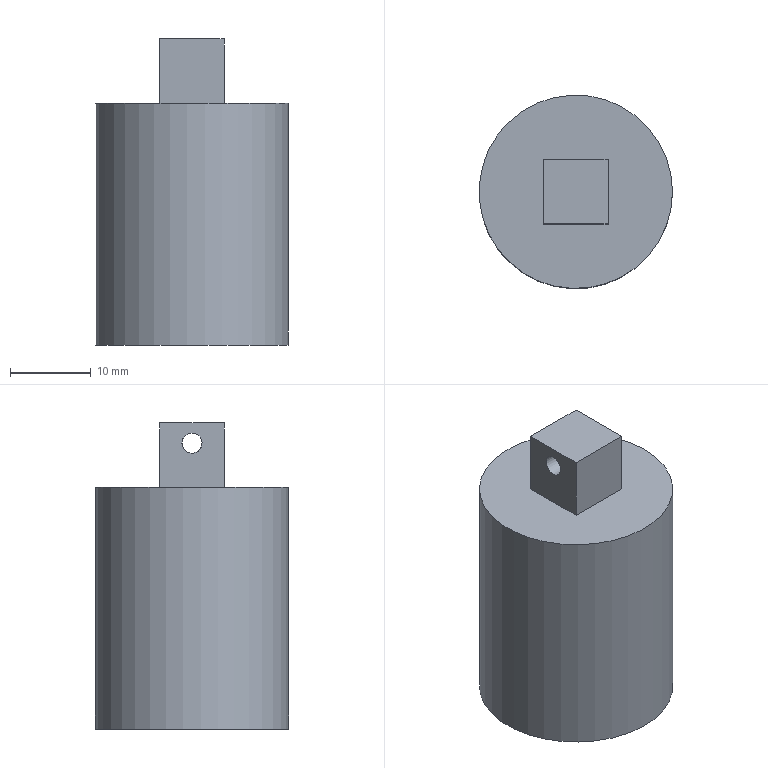Component | NX | ROBOT_ARM_BASE | 1 solid | 9 faces | box 24 x 24 x 38 mm | volume 14044 mm3 | plane 7 | cylinder 2 | commonest cylinder face diameters 24 x1 2.5 x1
STEP:
#1=CARTESIAN_POINT('',(0.,0.,0.));
#2=DIRECTION('',(0.,0.,1.));
#3=DIRECTION('',(1.,0.,0.));
#4=AXIS2_PLACEMENT_3D('',#1,#2,#3);
#5=CARTESIAN_POINT('',(23.471,13.498,36.));
#6=VERTEX_POINT('',#5);
#7=CARTESIAN_POINT('',(11.471,13.498,36.));
#8=DIRECTION('',(0.,0.,-1.));
#9=DIRECTION('',(1.,0.,0.));
#10=AXIS2_PLACEMENT_3D('',#7,#8,#9);
#11=CIRCLE('',#10,12.);
#12=CARTESIAN_POINT('',(11.471,13.498,36.));
#13=DIRECTION('',(0.,0.,-1.));
#14=DIRECTION('',(-1.,0.,0.));
#15=AXIS2_PLACEMENT_3D('',#12,#13,#14);
#16=PLANE('',#15);
#17=CARTESIAN_POINT('',(0.,0.));
#18=DIRECTION('',(-1.,0.));
#19=AXIS2_PLACEMENT_2D('',#17,#18);
#20=CIRCLE('',#19,12.);
#21=(GEOMETRIC_REPRESENTATION_CONTEXT(2)PARAMETRIC_REPRESENTATION_CONTEXT()REPRESENTATION_CONTEXT('',''));
#22=DEFINITIONAL_REPRESENTATION('',(#20),#21);
#23=PCURVE('',#16,#22);
#24=CARTESIAN_POINT('',(11.471,13.498,6.));
#25=DIRECTION('',(0.,0.,1.));
#26=DIRECTION('',(1.,0.,0.));
#27=AXIS2_PLACEMENT_3D('',#24,#25,#26);
#28=CYLINDRICAL_SURFACE('',#27,12.);
#29=CARTESIAN_POINT('',(6.283,30.));
#30=DIRECTION('',(-1.,0.));
#31=VECTOR('',#30,1.);
#32=LINE('',#29,#31);
#33=(GEOMETRIC_REPRESENTATION_CONTEXT(2)PARAMETRIC_REPRESENTATION_CONTEXT()REPRESENTATION_CONTEXT('',''));
#34=DEFINITIONAL_REPRESENTATION('',(#32),#33);
#35=PCURVE('',#28,#34);
#36=SURFACE_CURVE('',#11,(#23,#35),.PCURVE_S1.);
#37=EDGE_CURVE('',#6,#6,#36,.T.);
#38=ORIENTED_EDGE('',*,*,#37,.F.);
#39=EDGE_LOOP('',(#38));
#40=FACE_BOUND('',#39,.T.);
#41=CARTESIAN_POINT('',(7.471,17.498,36.));
#42=VERTEX_POINT('',#41);
#43=CARTESIAN_POINT('',(7.471,9.498,36.));
#44=VERTEX_POINT('',#43);
#45=CARTESIAN_POINT('',(7.471,17.498,36.));
#46=DIRECTION('',(-0.,-1.,0.));
#47=VECTOR('',#46,1.);
#48=LINE('',#45,#47);
#49=CARTESIAN_POINT('',(4.,4.));
#50=DIRECTION('',(0.,-1.));
#51=VECTOR('',#50,1.);
#52=LINE('',#49,#51);
#53=(GEOMETRIC_REPRESENTATION_CONTEXT(2)PARAMETRIC_REPRESENTATION_CONTEXT()REPRESENTATION_CONTEXT('',''));
#54=DEFINITIONAL_REPRESENTATION('',(#52),#53);
#55=PCURVE('',#16,#54);
#56=CARTESIAN_POINT('',(7.471,17.498,44.));
#57=DIRECTION('',(1.,-0.,0.));
#58=DIRECTION('',(0.,1.,0.));
#59=AXIS2_PLACEMENT_3D('',#56,#57,#58);
#60=PLANE('',#59);
#61=CARTESIAN_POINT('',(0.,-8.));
#62=DIRECTION('',(-1.,0.));
#63=VECTOR('',#62,1.);
#64=LINE('',#61,#63);
#65=(GEOMETRIC_REPRESENTATION_CONTEXT(2)PARAMETRIC_REPRESENTATION_CONTEXT()REPRESENTATION_CONTEXT('',''));
#66=DEFINITIONAL_REPRESENTATION('',(#64),#65);
#67=PCURVE('',#60,#66);
#68=SURFACE_CURVE('',#48,(#55,#67),.PCURVE_S1.);
#69=EDGE_CURVE('',#42,#44,#68,.T.);
#70=ORIENTED_EDGE('',*,*,#69,.F.);
#71=CARTESIAN_POINT('',(15.471,17.498,36.));
#72=VERTEX_POINT('',#71);
#73=CARTESIAN_POINT('',(15.471,17.498,36.));
#74=DIRECTION('',(-1.,0.,0.));
#75=VECTOR('',#74,1.);
#76=LINE('',#73,#75);
#77=CARTESIAN_POINT('',(-4.,4.));
#78=DIRECTION('',(1.,0.));
#79=VECTOR('',#78,1.);
#80=LINE('',#77,#79);
#81=(GEOMETRIC_REPRESENTATION_CONTEXT(2)PARAMETRIC_REPRESENTATION_CONTEXT()REPRESENTATION_CONTEXT('',''));
#82=DEFINITIONAL_REPRESENTATION('',(#80),#81);
#83=PCURVE('',#16,#82);
#84=CARTESIAN_POINT('',(15.471,17.498,44.));
#85=DIRECTION('',(-0.,-1.,0.));
#86=DIRECTION('',(1.,-0.,0.));
#87=AXIS2_PLACEMENT_3D('',#84,#85,#86);
#88=PLANE('',#87);
#89=CARTESIAN_POINT('',(0.,-8.));
#90=DIRECTION('',(-1.,0.));
#91=VECTOR('',#90,1.);
#92=LINE('',#89,#91);
#93=(GEOMETRIC_REPRESENTATION_CONTEXT(2)PARAMETRIC_REPRESENTATION_CONTEXT()REPRESENTATION_CONTEXT('',''));
#94=DEFINITIONAL_REPRESENTATION('',(#92),#93);
#95=PCURVE('',#88,#94);
#96=SURFACE_CURVE('',#76,(#83,#95),.PCURVE_S1.);
#97=EDGE_CURVE('',#72,#42,#96,.T.);
#98=ORIENTED_EDGE('',*,*,#97,.F.);
#99=CARTESIAN_POINT('',(15.471,9.498,36.));
#100=VERTEX_POINT('',#99);
#101=CARTESIAN_POINT('',(15.471,9.498,36.));
#102=DIRECTION('',(0.,1.,0.));
#103=VECTOR('',#102,1.);
#104=LINE('',#101,#103);
#105=CARTESIAN_POINT('',(-4.,-4.));
#106=DIRECTION('',(0.,1.));
#107=VECTOR('',#106,1.);
#108=LINE('',#105,#107);
#109=(GEOMETRIC_REPRESENTATION_CONTEXT(2)PARAMETRIC_REPRESENTATION_CONTEXT()REPRESENTATION_CONTEXT('',''));
#110=DEFINITIONAL_REPRESENTATION('',(#108),#109);
#111=PCURVE('',#16,#110);
#112=CARTESIAN_POINT('',(15.471,9.498,44.));
#113=DIRECTION('',(-1.,0.,0.));
#114=DIRECTION('',(0.,0.,1.));
#115=AXIS2_PLACEMENT_3D('',#112,#113,#114);
#116=PLANE('',#115);
#117=CARTESIAN_POINT('',(-8.,0.));
#118=DIRECTION('',(0.,1.));
#119=VECTOR('',#118,1.);
#120=LINE('',#117,#119);
#121=(GEOMETRIC_REPRESENTATION_CONTEXT(2)PARAMETRIC_REPRESENTATION_CONTEXT()REPRESENTATION_CONTEXT('',''));
#122=DEFINITIONAL_REPRESENTATION('',(#120),#121);
#123=PCURVE('',#116,#122);
#124=SURFACE_CURVE('',#104,(#111,#123),.PCURVE_S1.);
#125=EDGE_CURVE('',#100,#72,#124,.T.);
#126=ORIENTED_EDGE('',*,*,#125,.F.);
#127=CARTESIAN_POINT('',(7.471,9.498,36.));
#128=DIRECTION('',(1.,0.,0.));
#129=VECTOR('',#128,1.);
#130=LINE('',#127,#129);
#131=CARTESIAN_POINT('',(4.,-4.));
#132=DIRECTION('',(-1.,0.));
#133=VECTOR('',#132,1.);
#134=LINE('',#131,#133);
#135=(GEOMETRIC_REPRESENTATION_CONTEXT(2)PARAMETRIC_REPRESENTATION_CONTEXT()REPRESENTATION_CONTEXT('',''));
#136=DEFINITIONAL_REPRESENTATION('',(#134),#135);
#137=PCURVE('',#16,#136);
#138=CARTESIAN_POINT('',(7.471,9.498,44.));
#139=DIRECTION('',(0.,1.,0.));
#140=DIRECTION('',(0.,0.,1.));
#141=AXIS2_PLACEMENT_3D('',#138,#139,#140);
#142=PLANE('',#141);
#143=CARTESIAN_POINT('',(-8.,0.));
#144=DIRECTION('',(0.,1.));
#145=VECTOR('',#144,1.);
#146=LINE('',#143,#145);
#147=(GEOMETRIC_REPRESENTATION_CONTEXT(2)PARAMETRIC_REPRESENTATION_CONTEXT()REPRESENTATION_CONTEXT('',''));
#148=DEFINITIONAL_REPRESENTATION('',(#146),#147);
#149=PCURVE('',#142,#148);
#150=SURFACE_CURVE('',#130,(#137,#149),.PCURVE_S1.);
#151=EDGE_CURVE('',#44,#100,#150,.T.);
#152=ORIENTED_EDGE('',*,*,#151,.F.);
#153=EDGE_LOOP('',(#70,#98,#126,#152));
#154=FACE_BOUND('',#153,.T.);
#155=ADVANCED_FACE('',(#40,#154),#16,.F.);
#156=CARTESIAN_POINT('',(23.471,13.498,6.));
#157=VERTEX_POINT('',#156);
#158=CARTESIAN_POINT('',(11.471,13.498,6.));
#159=DIRECTION('',(0.,0.,-1.));
#160=DIRECTION('',(1.,0.,0.));
#161=AXIS2_PLACEMENT_3D('',#158,#159,#160);
#162=CIRCLE('',#161,12.);
#163=CARTESIAN_POINT('',(6.283,0.));
#164=DIRECTION('',(-1.,0.));
#165=VECTOR('',#164,1.);
#166=LINE('',#163,#165);
#167=(GEOMETRIC_REPRESENTATION_CONTEXT(2)PARAMETRIC_REPRESENTATION_CONTEXT()REPRESENTATION_CONTEXT('',''));
#168=DEFINITIONAL_REPRESENTATION('',(#166),#167);
#169=PCURVE('',#28,#168);
#170=CARTESIAN_POINT('',(11.471,13.498,6.));
#171=DIRECTION('',(0.,0.,-1.));
#172=DIRECTION('',(-1.,0.,0.));
#173=AXIS2_PLACEMENT_3D('',#170,#171,#172);
#174=PLANE('',#173);
#175=CARTESIAN_POINT('',(0.,0.));
#176=DIRECTION('',(-1.,0.));
#177=AXIS2_PLACEMENT_2D('',#175,#176);
#178=CIRCLE('',#177,12.);
#179=(GEOMETRIC_REPRESENTATION_CONTEXT(2)PARAMETRIC_REPRESENTATION_CONTEXT()REPRESENTATION_CONTEXT('',''));
#180=DEFINITIONAL_REPRESENTATION('',(#178),#179);
#181=PCURVE('',#174,#180);
#182=SURFACE_CURVE('',#162,(#169,#181),.PCURVE_S1.);
#183=EDGE_CURVE('',#157,#157,#182,.T.);
#184=ORIENTED_EDGE('',*,*,#183,.F.);
#185=CARTESIAN_POINT('',(23.471,13.498,6.));
#186=CARTESIAN_POINT('',(23.471,13.498,36.));
#187=B_SPLINE_CURVE_WITH_KNOTS('',1,(#185,#186),.UNSPECIFIED.,.F.,.F.,(2,2),(0.,30.),.PIECEWISE_BEZIER_KNOTS.);
#188=CARTESIAN_POINT('',(6.283,0.));
#189=DIRECTION('',(0.,1.));
#190=VECTOR('',#189,1.);
#191=LINE('',#188,#190);
#192=(GEOMETRIC_REPRESENTATION_CONTEXT(2)PARAMETRIC_REPRESENTATION_CONTEXT()REPRESENTATION_CONTEXT('',''));
#193=DEFINITIONAL_REPRESENTATION('',(#191),#192);
#194=PCURVE('',#28,#193);
#195=CARTESIAN_POINT('',(0.,0.));
#196=DIRECTION('',(0.,1.));
#197=VECTOR('',#196,1.);
#198=LINE('',#195,#197);
#199=(GEOMETRIC_REPRESENTATION_CONTEXT(2)PARAMETRIC_REPRESENTATION_CONTEXT()REPRESENTATION_CONTEXT('',''));
#200=DEFINITIONAL_REPRESENTATION('',(#198),#199);
#201=PCURVE('',#28,#200);
#202=SEAM_CURVE('',#187,(#194,#201),.PCURVE_S1.);
#203=EDGE_CURVE('',#157,#6,#202,.T.);
#204=ORIENTED_EDGE('',*,*,#203,.T.);
#205=ORIENTED_EDGE('',*,*,#37,.T.);
#206=ORIENTED_EDGE('',*,*,#203,.F.);
#207=EDGE_LOOP('',(#184,#204,#205,#206));
#208=FACE_BOUND('',#207,.T.);
#209=ADVANCED_FACE('',(#208),#28,.T.);
#210=ORIENTED_EDGE('',*,*,#183,.T.);
#211=EDGE_LOOP('',(#210));
#212=FACE_BOUND('',#211,.T.);
#213=ADVANCED_FACE('',(#212),#174,.T.);
#214=CARTESIAN_POINT('',(7.471,14.748,41.5));
#215=VERTEX_POINT('',#214);
#216=CARTESIAN_POINT('',(7.471,13.498,42.75));
#217=VERTEX_POINT('',#216);
#218=CARTESIAN_POINT('',(7.471,13.498,41.5));
#219=DIRECTION('',(-1.,0.,0.));
#220=DIRECTION('',(0.,1.,0.));
#221=AXIS2_PLACEMENT_3D('',#218,#219,#220);
#222=CIRCLE('',#221,1.25);
#223=CARTESIAN_POINT('',(-2.75,-2.5));
#224=CARTESIAN_POINT('',(-2.75,-4.665));
#225=CARTESIAN_POINT('',(-4.625,-3.583));
#226=CARTESIAN_POINT('',(-6.5,-2.5));
#227=CARTESIAN_POINT('',(-4.625,-1.417));
#228=CARTESIAN_POINT('',(-2.75,-0.3349));
#229=CARTESIAN_POINT('',(-2.75,-2.5));
#230=(BOUNDED_CURVE()B_SPLINE_CURVE(2,(#223,#224,#225,#226,#227,#228,#229),.UNSPECIFIED.,.T.,.F.)B_SPLINE_CURVE_WITH_KNOTS((1,2,2,2,2,1),(-2.094,0.,2.094,4.189,6.283,8.378),.UNSPECIFIED.)CURVE()GEOMETRIC_REPRESENTATION_ITEM()RATIONAL_B_SPLINE_CURVE((1.,0.5,1.,0.5,1.,0.5,1.))REPRESENTATION_ITEM(''));
#231=(GEOMETRIC_REPRESENTATION_CONTEXT(2)PARAMETRIC_REPRESENTATION_CONTEXT()REPRESENTATION_CONTEXT('',''));
#232=DEFINITIONAL_REPRESENTATION('',(#230),#231);
#233=PCURVE('',#60,#232);
#234=CARTESIAN_POINT('',(23.471,13.498,41.5));
#235=DIRECTION('',(-1.,0.,0.));
#236=DIRECTION('',(0.,0.,1.));
#237=AXIS2_PLACEMENT_3D('',#234,#235,#236);
#238=CYLINDRICAL_SURFACE('',#237,1.25);
#239=CARTESIAN_POINT('',(1.571,16.));
#240=DIRECTION('',(1.,0.));
#241=VECTOR('',#240,1.);
#242=LINE('',#239,#241);
#243=(GEOMETRIC_REPRESENTATION_CONTEXT(2)PARAMETRIC_REPRESENTATION_CONTEXT()REPRESENTATION_CONTEXT('',''));
#244=DEFINITIONAL_REPRESENTATION('',(#242),#243);
#245=PCURVE('',#238,#244);
#246=SURFACE_CURVE('',#222,(#233,#245),.PCURVE_S1.);
#247=EDGE_CURVE('',#215,#217,#246,.T.);
#248=ORIENTED_EDGE('',*,*,#247,.F.);
#249=CARTESIAN_POINT('',(7.471,13.498,41.5));
#250=DIRECTION('',(-1.,0.,0.));
#251=DIRECTION('',(0.,1.,0.));
#252=AXIS2_PLACEMENT_3D('',#249,#250,#251);
#253=CIRCLE('',#252,1.25);
#254=CARTESIAN_POINT('',(-2.75,-2.5));
#255=CARTESIAN_POINT('',(-2.75,-4.665));
#256=CARTESIAN_POINT('',(-4.625,-3.583));
#257=CARTESIAN_POINT('',(-6.5,-2.5));
#258=CARTESIAN_POINT('',(-4.625,-1.417));
#259=CARTESIAN_POINT('',(-2.75,-0.3349));
#260=CARTESIAN_POINT('',(-2.75,-2.5));
#261=(BOUNDED_CURVE()B_SPLINE_CURVE(2,(#254,#255,#256,#257,#258,#259,#260),.UNSPECIFIED.,.T.,.F.)B_SPLINE_CURVE_WITH_KNOTS((1,2,2,2,2,1),(-2.094,0.,2.094,4.189,6.283,8.378),.UNSPECIFIED.)CURVE()GEOMETRIC_REPRESENTATION_ITEM()RATIONAL_B_SPLINE_CURVE((1.,0.5,1.,0.5,1.,0.5,1.))REPRESENTATION_ITEM(''));
#262=(GEOMETRIC_REPRESENTATION_CONTEXT(2)PARAMETRIC_REPRESENTATION_CONTEXT()REPRESENTATION_CONTEXT('',''));
#263=DEFINITIONAL_REPRESENTATION('',(#261),#262);
#264=PCURVE('',#60,#263);
#265=CARTESIAN_POINT('',(-4.712,16.));
#266=DIRECTION('',(1.,0.));
#267=VECTOR('',#266,1.);
#268=LINE('',#265,#267);
#269=(GEOMETRIC_REPRESENTATION_CONTEXT(2)PARAMETRIC_REPRESENTATION_CONTEXT()REPRESENTATION_CONTEXT('',''));
#270=DEFINITIONAL_REPRESENTATION('',(#268),#269);
#271=PCURVE('',#238,#270);
#272=SURFACE_CURVE('',#253,(#264,#271),.PCURVE_S1.);
#273=EDGE_CURVE('',#217,#215,#272,.T.);
#274=ORIENTED_EDGE('',*,*,#273,.F.);
#275=EDGE_LOOP('',(#248,#274));
#276=FACE_BOUND('',#275,.T.);
#277=ORIENTED_EDGE('',*,*,#69,.T.);
#278=CARTESIAN_POINT('',(7.471,9.498,44.));
#279=VERTEX_POINT('',#278);
#280=CARTESIAN_POINT('',(7.471,9.498,44.));
#281=DIRECTION('',(0.,0.,-1.));
#282=VECTOR('',#281,1.);
#283=LINE('',#280,#282);
#284=CARTESIAN_POINT('',(-8.,0.));
#285=DIRECTION('',(0.,-1.));
#286=VECTOR('',#285,1.);
#287=LINE('',#284,#286);
#288=(GEOMETRIC_REPRESENTATION_CONTEXT(2)PARAMETRIC_REPRESENTATION_CONTEXT()REPRESENTATION_CONTEXT('',''));
#289=DEFINITIONAL_REPRESENTATION('',(#287),#288);
#290=PCURVE('',#60,#289);
#291=CARTESIAN_POINT('',(0.,0.));
#292=DIRECTION('',(-1.,0.));
#293=VECTOR('',#292,1.);
#294=LINE('',#291,#293);
#295=(GEOMETRIC_REPRESENTATION_CONTEXT(2)PARAMETRIC_REPRESENTATION_CONTEXT()REPRESENTATION_CONTEXT('',''));
#296=DEFINITIONAL_REPRESENTATION('',(#294),#295);
#297=PCURVE('',#142,#296);
#298=SURFACE_CURVE('',#283,(#290,#297),.PCURVE_S1.);
#299=EDGE_CURVE('',#279,#44,#298,.T.);
#300=ORIENTED_EDGE('',*,*,#299,.F.);
#301=CARTESIAN_POINT('',(7.471,17.498,44.));
#302=VERTEX_POINT('',#301);
#303=CARTESIAN_POINT('',(7.471,17.498,44.));
#304=DIRECTION('',(-0.,-1.,0.));
#305=VECTOR('',#304,1.);
#306=LINE('',#303,#305);
#307=CARTESIAN_POINT('',(0.,0.));
#308=DIRECTION('',(-1.,0.));
#309=VECTOR('',#308,1.);
#310=LINE('',#307,#309);
#311=(GEOMETRIC_REPRESENTATION_CONTEXT(2)PARAMETRIC_REPRESENTATION_CONTEXT()REPRESENTATION_CONTEXT('',''));
#312=DEFINITIONAL_REPRESENTATION('',(#310),#311);
#313=PCURVE('',#60,#312);
#314=CARTESIAN_POINT('',(11.471,13.498,44.));
#315=DIRECTION('',(0.,0.,1.));
#316=DIRECTION('',(1.,0.,0.));
#317=AXIS2_PLACEMENT_3D('',#314,#315,#316);
#318=PLANE('',#317);
#319=CARTESIAN_POINT('',(-4.,4.));
#320=DIRECTION('',(-0.,-1.));
#321=VECTOR('',#320,1.);
#322=LINE('',#319,#321);
#323=(GEOMETRIC_REPRESENTATION_CONTEXT(2)PARAMETRIC_REPRESENTATION_CONTEXT()REPRESENTATION_CONTEXT('',''));
#324=DEFINITIONAL_REPRESENTATION('',(#322),#323);
#325=PCURVE('',#318,#324);
#326=SURFACE_CURVE('',#306,(#313,#325),.PCURVE_S1.);
#327=EDGE_CURVE('',#302,#279,#326,.T.);
#328=ORIENTED_EDGE('',*,*,#327,.F.);
#329=CARTESIAN_POINT('',(7.471,17.498,44.));
#330=DIRECTION('',(0.,0.,-1.));
#331=VECTOR('',#330,1.);
#332=LINE('',#329,#331);
#333=CARTESIAN_POINT('',(0.,0.));
#334=DIRECTION('',(0.,-1.));
#335=VECTOR('',#334,1.);
#336=LINE('',#333,#335);
#337=(GEOMETRIC_REPRESENTATION_CONTEXT(2)PARAMETRIC_REPRESENTATION_CONTEXT()REPRESENTATION_CONTEXT('',''));
#338=DEFINITIONAL_REPRESENTATION('',(#336),#337);
#339=PCURVE('',#60,#338);
#340=CARTESIAN_POINT('',(-8.,0.));
#341=DIRECTION('',(0.,-1.));
#342=VECTOR('',#341,1.);
#343=LINE('',#340,#342);
#344=(GEOMETRIC_REPRESENTATION_CONTEXT(2)PARAMETRIC_REPRESENTATION_CONTEXT()REPRESENTATION_CONTEXT('',''));
#345=DEFINITIONAL_REPRESENTATION('',(#343),#344);
#346=PCURVE('',#88,#345);
#347=SURFACE_CURVE('',#332,(#339,#346),.PCURVE_S1.);
#348=EDGE_CURVE('',#302,#42,#347,.T.);
#349=ORIENTED_EDGE('',*,*,#348,.T.);
#350=EDGE_LOOP('',(#277,#300,#328,#349));
#351=FACE_BOUND('',#350,.T.);
#352=ADVANCED_FACE('',(#276,#351),#60,.F.);
#353=ORIENTED_EDGE('',*,*,#151,.T.);
#354=CARTESIAN_POINT('',(15.471,9.498,44.));
#355=VERTEX_POINT('',#354);
#356=CARTESIAN_POINT('',(15.471,9.498,44.));
#357=DIRECTION('',(0.,0.,-1.));
#358=VECTOR('',#357,1.);
#359=LINE('',#356,#358);
#360=CARTESIAN_POINT('',(0.,8.));
#361=DIRECTION('',(-1.,0.));
#362=VECTOR('',#361,1.);
#363=LINE('',#360,#362);
#364=(GEOMETRIC_REPRESENTATION_CONTEXT(2)PARAMETRIC_REPRESENTATION_CONTEXT()REPRESENTATION_CONTEXT('',''));
#365=DEFINITIONAL_REPRESENTATION('',(#363),#364);
#366=PCURVE('',#142,#365);
#367=CARTESIAN_POINT('',(0.,0.));
#368=DIRECTION('',(-1.,0.));
#369=VECTOR('',#368,1.);
#370=LINE('',#367,#369);
#371=(GEOMETRIC_REPRESENTATION_CONTEXT(2)PARAMETRIC_REPRESENTATION_CONTEXT()REPRESENTATION_CONTEXT('',''));
#372=DEFINITIONAL_REPRESENTATION('',(#370),#371);
#373=PCURVE('',#116,#372);
#374=SURFACE_CURVE('',#359,(#366,#373),.PCURVE_S1.);
#375=EDGE_CURVE('',#355,#100,#374,.T.);
#376=ORIENTED_EDGE('',*,*,#375,.F.);
#377=CARTESIAN_POINT('',(7.471,9.498,44.));
#378=DIRECTION('',(1.,0.,0.));
#379=VECTOR('',#378,1.);
#380=LINE('',#377,#379);
#381=CARTESIAN_POINT('',(0.,0.));
#382=DIRECTION('',(0.,1.));
#383=VECTOR('',#382,1.);
#384=LINE('',#381,#383);
#385=(GEOMETRIC_REPRESENTATION_CONTEXT(2)PARAMETRIC_REPRESENTATION_CONTEXT()REPRESENTATION_CONTEXT('',''));
#386=DEFINITIONAL_REPRESENTATION('',(#384),#385);
#387=PCURVE('',#142,#386);
#388=CARTESIAN_POINT('',(-4.,-4.));
#389=DIRECTION('',(1.,0.));
#390=VECTOR('',#389,1.);
#391=LINE('',#388,#390);
#392=(GEOMETRIC_REPRESENTATION_CONTEXT(2)PARAMETRIC_REPRESENTATION_CONTEXT()REPRESENTATION_CONTEXT('',''));
#393=DEFINITIONAL_REPRESENTATION('',(#391),#392);
#394=PCURVE('',#318,#393);
#395=SURFACE_CURVE('',#380,(#387,#394),.PCURVE_S1.);
#396=EDGE_CURVE('',#279,#355,#395,.T.);
#397=ORIENTED_EDGE('',*,*,#396,.F.);
#398=ORIENTED_EDGE('',*,*,#299,.T.);
#399=EDGE_LOOP('',(#353,#376,#397,#398));
#400=FACE_BOUND('',#399,.T.);
#401=ADVANCED_FACE('',(#400),#142,.F.);
#402=CARTESIAN_POINT('',(15.471,13.498,42.75));
#403=VERTEX_POINT('',#402);
#404=CARTESIAN_POINT('',(15.471,13.498,41.5));
#405=DIRECTION('',(1.,0.,0.));
#406=DIRECTION('',(0.,0.,1.));
#407=AXIS2_PLACEMENT_3D('',#404,#405,#406);
#408=CIRCLE('',#407,1.25);
#409=CARTESIAN_POINT('',(-1.25,4.));
#410=CARTESIAN_POINT('',(-1.25,1.835));
#411=CARTESIAN_POINT('',(-3.125,2.917));
#412=CARTESIAN_POINT('',(-5.,4.));
#413=CARTESIAN_POINT('',(-3.125,5.083));
#414=CARTESIAN_POINT('',(-1.25,6.165));
#415=CARTESIAN_POINT('',(-1.25,4.));
#416=(BOUNDED_CURVE()B_SPLINE_CURVE(2,(#409,#410,#411,#412,#413,#414,#415),.UNSPECIFIED.,.T.,.F.)B_SPLINE_CURVE_WITH_KNOTS((1,2,2,2,2,1),(-2.094,0.,2.094,4.189,6.283,8.378),.UNSPECIFIED.)CURVE()GEOMETRIC_REPRESENTATION_ITEM()RATIONAL_B_SPLINE_CURVE((1.,0.5,1.,0.5,1.,0.5,1.))REPRESENTATION_ITEM(''));
#417=(GEOMETRIC_REPRESENTATION_CONTEXT(2)PARAMETRIC_REPRESENTATION_CONTEXT()REPRESENTATION_CONTEXT('',''));
#418=DEFINITIONAL_REPRESENTATION('',(#416),#417);
#419=PCURVE('',#116,#418);
#420=CARTESIAN_POINT('',(6.283,8.));
#421=DIRECTION('',(-1.,0.));
#422=VECTOR('',#421,1.);
#423=LINE('',#420,#422);
#424=(GEOMETRIC_REPRESENTATION_CONTEXT(2)PARAMETRIC_REPRESENTATION_CONTEXT()REPRESENTATION_CONTEXT('',''));
#425=DEFINITIONAL_REPRESENTATION('',(#423),#424);
#426=PCURVE('',#238,#425);
#427=SURFACE_CURVE('',#408,(#419,#426),.PCURVE_S1.);
#428=EDGE_CURVE('',#403,#403,#427,.T.);
#429=ORIENTED_EDGE('',*,*,#428,.F.);
#430=EDGE_LOOP('',(#429));
#431=FACE_BOUND('',#430,.T.);
#432=ORIENTED_EDGE('',*,*,#125,.T.);
#433=CARTESIAN_POINT('',(15.471,17.498,44.));
#434=VERTEX_POINT('',#433);
#435=CARTESIAN_POINT('',(15.471,17.498,44.));
#436=DIRECTION('',(0.,0.,-1.));
#437=VECTOR('',#436,1.);
#438=LINE('',#435,#437);
#439=CARTESIAN_POINT('',(0.,8.));
#440=DIRECTION('',(-1.,0.));
#441=VECTOR('',#440,1.);
#442=LINE('',#439,#441);
#443=(GEOMETRIC_REPRESENTATION_CONTEXT(2)PARAMETRIC_REPRESENTATION_CONTEXT()REPRESENTATION_CONTEXT('',''));
#444=DEFINITIONAL_REPRESENTATION('',(#442),#443);
#445=PCURVE('',#116,#444);
#446=CARTESIAN_POINT('',(0.,0.));
#447=DIRECTION('',(0.,-1.));
#448=VECTOR('',#447,1.);
#449=LINE('',#446,#448);
#450=(GEOMETRIC_REPRESENTATION_CONTEXT(2)PARAMETRIC_REPRESENTATION_CONTEXT()REPRESENTATION_CONTEXT('',''));
#451=DEFINITIONAL_REPRESENTATION('',(#449),#450);
#452=PCURVE('',#88,#451);
#453=SURFACE_CURVE('',#438,(#445,#452),.PCURVE_S1.);
#454=EDGE_CURVE('',#434,#72,#453,.T.);
#455=ORIENTED_EDGE('',*,*,#454,.F.);
#456=CARTESIAN_POINT('',(15.471,9.498,44.));
#457=DIRECTION('',(0.,1.,0.));
#458=VECTOR('',#457,1.);
#459=LINE('',#456,#458);
#460=CARTESIAN_POINT('',(0.,0.));
#461=DIRECTION('',(0.,1.));
#462=VECTOR('',#461,1.);
#463=LINE('',#460,#462);
#464=(GEOMETRIC_REPRESENTATION_CONTEXT(2)PARAMETRIC_REPRESENTATION_CONTEXT()REPRESENTATION_CONTEXT('',''));
#465=DEFINITIONAL_REPRESENTATION('',(#463),#464);
#466=PCURVE('',#116,#465);
#467=CARTESIAN_POINT('',(4.,-4.));
#468=DIRECTION('',(0.,1.));
#469=VECTOR('',#468,1.);
#470=LINE('',#467,#469);
#471=(GEOMETRIC_REPRESENTATION_CONTEXT(2)PARAMETRIC_REPRESENTATION_CONTEXT()REPRESENTATION_CONTEXT('',''));
#472=DEFINITIONAL_REPRESENTATION('',(#470),#471);
#473=PCURVE('',#318,#472);
#474=SURFACE_CURVE('',#459,(#466,#473),.PCURVE_S1.);
#475=EDGE_CURVE('',#355,#434,#474,.T.);
#476=ORIENTED_EDGE('',*,*,#475,.F.);
#477=ORIENTED_EDGE('',*,*,#375,.T.);
#478=EDGE_LOOP('',(#432,#455,#476,#477));
#479=FACE_BOUND('',#478,.T.);
#480=ADVANCED_FACE('',(#431,#479),#116,.F.);
#481=ORIENTED_EDGE('',*,*,#97,.T.);
#482=ORIENTED_EDGE('',*,*,#348,.F.);
#483=CARTESIAN_POINT('',(15.471,17.498,44.));
#484=DIRECTION('',(-1.,0.,0.));
#485=VECTOR('',#484,1.);
#486=LINE('',#483,#485);
#487=CARTESIAN_POINT('',(0.,0.));
#488=DIRECTION('',(-1.,0.));
#489=VECTOR('',#488,1.);
#490=LINE('',#487,#489);
#491=(GEOMETRIC_REPRESENTATION_CONTEXT(2)PARAMETRIC_REPRESENTATION_CONTEXT()REPRESENTATION_CONTEXT('',''));
#492=DEFINITIONAL_REPRESENTATION('',(#490),#491);
#493=PCURVE('',#88,#492);
#494=CARTESIAN_POINT('',(4.,4.));
#495=DIRECTION('',(-1.,0.));
#496=VECTOR('',#495,1.);
#497=LINE('',#494,#496);
#498=(GEOMETRIC_REPRESENTATION_CONTEXT(2)PARAMETRIC_REPRESENTATION_CONTEXT()REPRESENTATION_CONTEXT('',''));
#499=DEFINITIONAL_REPRESENTATION('',(#497),#498);
#500=PCURVE('',#318,#499);
#501=SURFACE_CURVE('',#486,(#493,#500),.PCURVE_S1.);
#502=EDGE_CURVE('',#434,#302,#501,.T.);
#503=ORIENTED_EDGE('',*,*,#502,.F.);
#504=ORIENTED_EDGE('',*,*,#454,.T.);
#505=EDGE_LOOP('',(#481,#482,#503,#504));
#506=FACE_BOUND('',#505,.T.);
#507=ADVANCED_FACE('',(#506),#88,.F.);
#508=ORIENTED_EDGE('',*,*,#327,.T.);
#509=ORIENTED_EDGE('',*,*,#396,.T.);
#510=ORIENTED_EDGE('',*,*,#475,.T.);
#511=ORIENTED_EDGE('',*,*,#502,.T.);
#512=EDGE_LOOP('',(#508,#509,#510,#511));
#513=FACE_BOUND('',#512,.T.);
#514=ADVANCED_FACE('',(#513),#318,.T.);
#515=ORIENTED_EDGE('',*,*,#428,.F.);
#516=CARTESIAN_POINT('',(15.471,13.498,42.75));
#517=CARTESIAN_POINT('',(7.471,13.498,42.75));
#518=B_SPLINE_CURVE_WITH_KNOTS('',1,(#516,#517),.UNSPECIFIED.,.F.,.F.,(2,2),(8.,16.),.PIECEWISE_BEZIER_KNOTS.);
#519=CARTESIAN_POINT('',(6.283,0.));
#520=DIRECTION('',(0.,1.));
#521=VECTOR('',#520,1.);
#522=LINE('',#519,#521);
#523=(GEOMETRIC_REPRESENTATION_CONTEXT(2)PARAMETRIC_REPRESENTATION_CONTEXT()REPRESENTATION_CONTEXT('',''));
#524=DEFINITIONAL_REPRESENTATION('',(#522),#523);
#525=PCURVE('',#238,#524);
#526=CARTESIAN_POINT('',(0.,0.));
#527=DIRECTION('',(0.,1.));
#528=VECTOR('',#527,1.);
#529=LINE('',#526,#528);
#530=(GEOMETRIC_REPRESENTATION_CONTEXT(2)PARAMETRIC_REPRESENTATION_CONTEXT()REPRESENTATION_CONTEXT('',''));
#531=DEFINITIONAL_REPRESENTATION('',(#529),#530);
#532=PCURVE('',#238,#531);
#533=SEAM_CURVE('',#518,(#525,#532),.PCURVE_S1.);
#534=EDGE_CURVE('',#403,#217,#533,.T.);
#535=ORIENTED_EDGE('',*,*,#534,.T.);
#536=ORIENTED_EDGE('',*,*,#247,.F.);
#537=ORIENTED_EDGE('',*,*,#273,.F.);
#538=ORIENTED_EDGE('',*,*,#534,.F.);
#539=EDGE_LOOP('',(#515,#535,#536,#537,#538));
#540=FACE_BOUND('',#539,.F.);
#541=ADVANCED_FACE('',(#540),#238,.F.);
#542=CLOSED_SHELL('',(#155,#209,#213,#352,#401,#480,#507,#514,#541));
#543=MANIFOLD_SOLID_BREP('',#542);
#544=(LENGTH_UNIT()NAMED_UNIT(*)SI_UNIT(.MILLI.,.METRE.));
#545=UNCERTAINTY_MEASURE_WITH_UNIT(LENGTH_MEASURE(0.000002),#544,'','');
#546=(NAMED_UNIT(*)PLANE_ANGLE_UNIT()SI_UNIT($,.RADIAN.));
#547=(NAMED_UNIT(*)SI_UNIT($,.STERADIAN.)SOLID_ANGLE_UNIT());
#548=(GEOMETRIC_REPRESENTATION_CONTEXT(3)GLOBAL_UNCERTAINTY_ASSIGNED_CONTEXT((#545))GLOBAL_UNIT_ASSIGNED_CONTEXT((#544,#546,#547))REPRESENTATION_CONTEXT('',''));
#549=ADVANCED_BREP_SHAPE_REPRESENTATION('',(#4,#543),#548);